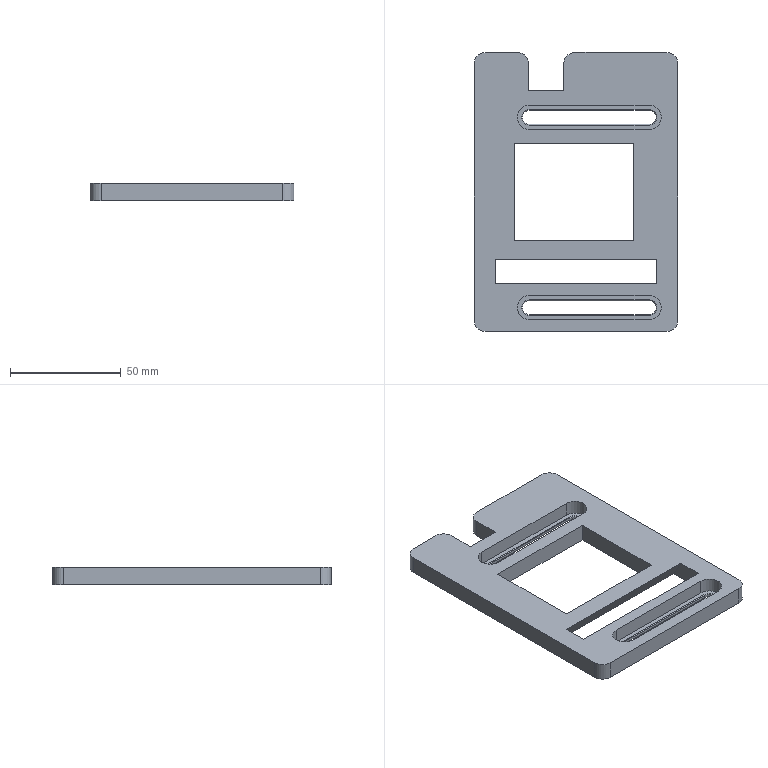Component | NX | MOUNTING_BRACKET | 1 solid | 50 faces | volume 53124 mm3 | plane 32 | cylinder 14 | cone 4 | commonest cylinder face diameters 10 x6 11 x4 6.4 x4